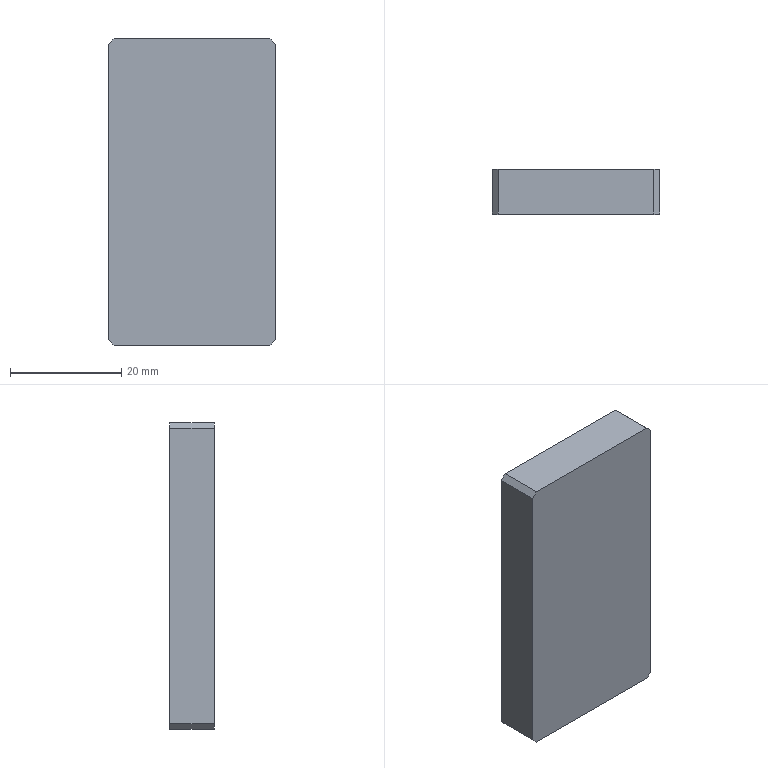Component | SolidWorks | GripperJaw1-1 | 1 solid | 16 faces | box 30 x 8 x 55 mm | volume 12147 mm3 | plane 14 | cylinder 2 | commonest cylinder face diameters 4 x2 | material 1060 Alloy
build123d program:
from build123d import *

# Parameters (mm, degrees)
SKETCH1_W           = 30
SKETCH1_H           = 55
BOSS_EXTRUDE1_DEPTH = 8
SKETCH2_W           = 20
SKETCH2_H           = 52
CUT_EXTRUDE1_DEPTH  = 2
FILLET1_R           = 2
CHAMFER1_SIZE       = 1


with BuildPart() as part:
    # Sketch1 → Boss-Extrude1 (new body)
    with BuildSketch(Plane.XY):
        Rectangle(SKETCH1_W, SKETCH1_H)
    extrude(amount=BOSS_EXTRUDE1_DEPTH)

    # Sketch2 → Cut-Extrude1 (cut)
    with BuildSketch(Plane.XY.offset(8)):
        with Locations((0, 27.5)):
            Rectangle(SKETCH2_W, SKETCH2_H)
    extrude(amount=-CUT_EXTRUDE1_DEPTH, mode=Mode.SUBTRACT)

    # Fillet1
    fillet1_edges = [part.edges().sort_by_distance(p)[0] for p in [
        (-10, 1.5, 7),
        (10, 1.5, 7),
    ]]
    fillet(fillet1_edges, radius=FILLET1_R)

    # Chamfer1
    chamfer1_edges = [part.edges().sort_by_distance(p)[0] for p in [
        (15, -27.5, 4),
        (-15, -27.5, 4),
        (-15, 27.5, 4),
        (15, 27.5, 4),
    ]]
    chamfer(chamfer1_edges, length=CHAMFER1_SIZE)


solid = part.part

# Placed as in the assembly
solid = solid.moved(Location((-45.188, -69.343, 163.22), (-90, 0, 0)))
STEP:
#1=COLOUR_RGB('',0.7922,0.8196,0.9333);
#2=FILL_AREA_STYLE_COLOUR('',#1);
#3=FILL_AREA_STYLE('',(#2));
#4=SURFACE_STYLE_FILL_AREA(#3);
#5=SURFACE_SIDE_STYLE('',(#4));
#6=SURFACE_STYLE_USAGE(.BOTH.,#5);
#7=PRESENTATION_STYLE_ASSIGNMENT((#6));
#8=CARTESIAN_POINT('',(-1.188,-2.415,7.469));
#9=VERTEX_POINT('',#8);
#10=CARTESIAN_POINT('',(-1.188,-2.415,5.383));
#11=VERTEX_POINT('',#10);
#12=CARTESIAN_POINT('',(-1.188,-2.415,5.343));
#13=DIRECTION('',(-0.,0.,-1.));
#14=VECTOR('',#13,39.37);
#15=LINE('',#12,#14);
#16=EDGE_CURVE('',#9,#11,#15,.T.);
#17=ORIENTED_EDGE('',*,*,#16,.F.);
#18=CARTESIAN_POINT('',(-1.188,-2.73,7.469));
#19=VERTEX_POINT('',#18);
#20=CARTESIAN_POINT('',(-1.188,-2.415,7.469));
#21=DIRECTION('',(0.,-1.,0.));
#22=VECTOR('',#21,39.37);
#23=LINE('',#20,#22);
#24=EDGE_CURVE('',#9,#19,#23,.T.);
#25=ORIENTED_EDGE('',*,*,#24,.T.);
#26=CARTESIAN_POINT('',(-1.188,-2.73,5.383));
#27=VERTEX_POINT('',#26);
#28=CARTESIAN_POINT('',(-1.188,-2.73,5.343));
#29=DIRECTION('',(-0.,0.,-1.));
#30=VECTOR('',#29,39.37);
#31=LINE('',#28,#30);
#32=EDGE_CURVE('',#19,#27,#31,.T.);
#33=ORIENTED_EDGE('',*,*,#32,.T.);
#34=CARTESIAN_POINT('',(-1.188,-2.415,5.383));
#35=DIRECTION('',(0.,1.,0.));
#36=VECTOR('',#35,39.37);
#37=LINE('',#34,#36);
#38=EDGE_CURVE('',#27,#11,#37,.T.);
#39=ORIENTED_EDGE('',*,*,#38,.T.);
#40=EDGE_LOOP('',(#17,#25,#33,#39));
#41=FACE_OUTER_BOUND('',#40,.T.);
#42=CARTESIAN_POINT('',(-1.188,-2.415,5.343));
#43=DIRECTION('',(-1.,0.,0.));
#44=DIRECTION('',(0.,0.,1.));
#45=AXIS2_PLACEMENT_3D('',#42,#43,#44);
#46=PLANE('',#45);
#47=ADVANCED_FACE('',(#41),#46,.F.);
#48=CARTESIAN_POINT('',(-1.228,-2.415,5.343));
#49=VERTEX_POINT('',#48);
#50=CARTESIAN_POINT('',(-1.385,-2.415,5.343));
#51=VERTEX_POINT('',#50);
#52=CARTESIAN_POINT('',(-2.37,-2.415,5.343));
#53=DIRECTION('',(-1.,0.,0.));
#54=VECTOR('',#53,39.37);
#55=LINE('',#52,#54);
#56=EDGE_CURVE('',#49,#51,#55,.T.);
#57=ORIENTED_EDGE('',*,*,#56,.F.);
#58=CARTESIAN_POINT('',(-1.228,-2.73,5.343));
#59=VERTEX_POINT('',#58);
#60=CARTESIAN_POINT('',(-1.228,-2.415,5.343));
#61=DIRECTION('',(0.,-1.,0.));
#62=VECTOR('',#61,39.37);
#63=LINE('',#60,#62);
#64=EDGE_CURVE('',#49,#59,#63,.T.);
#65=ORIENTED_EDGE('',*,*,#64,.T.);
#66=CARTESIAN_POINT('',(-2.33,-2.73,5.343));
#67=VERTEX_POINT('',#66);
#68=CARTESIAN_POINT('',(-2.37,-2.73,5.343));
#69=DIRECTION('',(-1.,0.,0.));
#70=VECTOR('',#69,39.37);
#71=LINE('',#68,#70);
#72=EDGE_CURVE('',#59,#67,#71,.T.);
#73=ORIENTED_EDGE('',*,*,#72,.T.);
#74=CARTESIAN_POINT('',(-2.33,-2.415,5.343));
#75=VERTEX_POINT('',#74);
#76=CARTESIAN_POINT('',(-2.33,-2.415,5.343));
#77=DIRECTION('',(0.,1.,0.));
#78=VECTOR('',#77,39.37);
#79=LINE('',#76,#78);
#80=EDGE_CURVE('',#67,#75,#79,.T.);
#81=ORIENTED_EDGE('',*,*,#80,.T.);
#82=CARTESIAN_POINT('',(-2.173,-2.415,5.343));
#83=VERTEX_POINT('',#82);
#84=CARTESIAN_POINT('',(-2.37,-2.415,5.343));
#85=DIRECTION('',(-1.,0.,0.));
#86=VECTOR('',#85,39.37);
#87=LINE('',#84,#86);
#88=EDGE_CURVE('',#83,#75,#87,.T.);
#89=ORIENTED_EDGE('',*,*,#88,.F.);
#90=CARTESIAN_POINT('',(-2.173,-2.494,5.343));
#91=VERTEX_POINT('',#90);
#92=CARTESIAN_POINT('',(-2.173,-2.415,5.343));
#93=DIRECTION('',(0.,-1.,0.));
#94=VECTOR('',#93,39.37);
#95=LINE('',#92,#94);
#96=EDGE_CURVE('',#83,#91,#95,.T.);
#97=ORIENTED_EDGE('',*,*,#96,.T.);
#98=CARTESIAN_POINT('',(-1.385,-2.494,5.343));
#99=VERTEX_POINT('',#98);
#100=CARTESIAN_POINT('',(-2.37,-2.494,5.343));
#101=DIRECTION('',(-1.,0.,0.));
#102=VECTOR('',#101,39.37);
#103=LINE('',#100,#102);
#104=EDGE_CURVE('',#99,#91,#103,.T.);
#105=ORIENTED_EDGE('',*,*,#104,.F.);
#106=CARTESIAN_POINT('',(-1.385,-2.415,5.343));
#107=DIRECTION('',(0.,1.,0.));
#108=VECTOR('',#107,39.37);
#109=LINE('',#106,#108);
#110=EDGE_CURVE('',#99,#51,#109,.T.);
#111=ORIENTED_EDGE('',*,*,#110,.T.);
#112=EDGE_LOOP('',(#57,#65,#73,#81,#89,#97,#105,#111));
#113=FACE_OUTER_BOUND('',#112,.T.);
#114=CARTESIAN_POINT('',(-2.37,-2.415,5.343));
#115=DIRECTION('',(0.,0.,1.));
#116=DIRECTION('',(0.,-1.,0.));
#117=AXIS2_PLACEMENT_3D('',#114,#115,#116);
#118=PLANE('',#117);
#119=ADVANCED_FACE('',(#113),#118,.F.);
#120=CARTESIAN_POINT('',(-2.37,-2.73,5.383));
#121=VERTEX_POINT('',#120);
#122=CARTESIAN_POINT('',(-2.37,-2.73,7.469));
#123=VERTEX_POINT('',#122);
#124=CARTESIAN_POINT('',(-2.37,-2.73,5.343));
#125=DIRECTION('',(0.,0.,1.));
#126=VECTOR('',#125,39.37);
#127=LINE('',#124,#126);
#128=EDGE_CURVE('',#121,#123,#127,.T.);
#129=ORIENTED_EDGE('',*,*,#128,.T.);
#130=CARTESIAN_POINT('',(-2.37,-2.415,7.469));
#131=VERTEX_POINT('',#130);
#132=CARTESIAN_POINT('',(-2.37,-2.415,7.469));
#133=DIRECTION('',(0.,1.,0.));
#134=VECTOR('',#133,39.37);
#135=LINE('',#132,#134);
#136=EDGE_CURVE('',#123,#131,#135,.T.);
#137=ORIENTED_EDGE('',*,*,#136,.T.);
#138=CARTESIAN_POINT('',(-2.37,-2.415,5.383));
#139=VERTEX_POINT('',#138);
#140=CARTESIAN_POINT('',(-2.37,-2.415,5.343));
#141=DIRECTION('',(0.,0.,1.));
#142=VECTOR('',#141,39.37);
#143=LINE('',#140,#142);
#144=EDGE_CURVE('',#139,#131,#143,.T.);
#145=ORIENTED_EDGE('',*,*,#144,.F.);
#146=CARTESIAN_POINT('',(-2.37,-2.415,5.383));
#147=DIRECTION('',(0.,-1.,0.));
#148=VECTOR('',#147,39.37);
#149=LINE('',#146,#148);
#150=EDGE_CURVE('',#139,#121,#149,.T.);
#151=ORIENTED_EDGE('',*,*,#150,.T.);
#152=EDGE_LOOP('',(#129,#137,#145,#151));
#153=FACE_OUTER_BOUND('',#152,.T.);
#154=CARTESIAN_POINT('',(-2.37,-2.415,5.343));
#155=DIRECTION('',(1.,0.,-0.));
#156=DIRECTION('',(-0.,0.,-1.));
#157=AXIS2_PLACEMENT_3D('',#154,#155,#156);
#158=PLANE('',#157);
#159=ADVANCED_FACE('',(#153),#158,.F.);
#160=CARTESIAN_POINT('',(-2.33,-2.73,7.509));
#161=VERTEX_POINT('',#160);
#162=CARTESIAN_POINT('',(-1.228,-2.73,7.509));
#163=VERTEX_POINT('',#162);
#164=CARTESIAN_POINT('',(-2.37,-2.73,7.509));
#165=DIRECTION('',(1.,0.,0.));
#166=VECTOR('',#165,39.37);
#167=LINE('',#164,#166);
#168=EDGE_CURVE('',#161,#163,#167,.T.);
#169=ORIENTED_EDGE('',*,*,#168,.T.);
#170=CARTESIAN_POINT('',(-1.228,-2.415,7.509));
#171=VERTEX_POINT('',#170);
#172=CARTESIAN_POINT('',(-1.228,-2.415,7.509));
#173=DIRECTION('',(0.,1.,0.));
#174=VECTOR('',#173,39.37);
#175=LINE('',#172,#174);
#176=EDGE_CURVE('',#163,#171,#175,.T.);
#177=ORIENTED_EDGE('',*,*,#176,.T.);
#178=CARTESIAN_POINT('',(-2.33,-2.415,7.509));
#179=VERTEX_POINT('',#178);
#180=CARTESIAN_POINT('',(-2.37,-2.415,7.509));
#181=DIRECTION('',(1.,0.,0.));
#182=VECTOR('',#181,39.37);
#183=LINE('',#180,#182);
#184=EDGE_CURVE('',#179,#171,#183,.T.);
#185=ORIENTED_EDGE('',*,*,#184,.F.);
#186=CARTESIAN_POINT('',(-2.33,-2.415,7.509));
#187=DIRECTION('',(0.,-1.,0.));
#188=VECTOR('',#187,39.37);
#189=LINE('',#186,#188);
#190=EDGE_CURVE('',#179,#161,#189,.T.);
#191=ORIENTED_EDGE('',*,*,#190,.T.);
#192=EDGE_LOOP('',(#169,#177,#185,#191));
#193=FACE_OUTER_BOUND('',#192,.T.);
#194=CARTESIAN_POINT('',(-2.37,-2.415,7.509));
#195=DIRECTION('',(0.,0.,-1.));
#196=DIRECTION('',(0.,1.,0.));
#197=AXIS2_PLACEMENT_3D('',#194,#195,#196);
#198=PLANE('',#197);
#199=ADVANCED_FACE('',(#193),#198,.F.);
#200=ORIENTED_EDGE('',*,*,#184,.T.);
#201=CARTESIAN_POINT('',(-0.9621,-2.415,7.243));
#202=DIRECTION('',(0.7071,0.,-0.7071));
#203=VECTOR('',#202,39.37);
#204=LINE('',#201,#203);
#205=EDGE_CURVE('',#171,#9,#204,.T.);
#206=ORIENTED_EDGE('',*,*,#205,.T.);
#207=ORIENTED_EDGE('',*,*,#16,.T.);
#208=CARTESIAN_POINT('',(-0.9621,-2.415,5.609));
#209=DIRECTION('',(-0.7071,0.,-0.7071));
#210=VECTOR('',#209,39.37);
#211=LINE('',#208,#210);
#212=EDGE_CURVE('',#11,#49,#211,.T.);
#213=ORIENTED_EDGE('',*,*,#212,.T.);
#214=ORIENTED_EDGE('',*,*,#56,.T.);
#215=CARTESIAN_POINT('',(-1.385,-2.415,6.288));
#216=VERTEX_POINT('',#215);
#217=CARTESIAN_POINT('',(-1.385,-2.415,4.32));
#218=DIRECTION('',(-0.,0.,-1.));
#219=VECTOR('',#218,39.37);
#220=LINE('',#217,#219);
#221=EDGE_CURVE('',#216,#51,#220,.T.);
#222=ORIENTED_EDGE('',*,*,#221,.F.);
#223=CARTESIAN_POINT('',(-1.464,-2.415,6.367));
#224=VERTEX_POINT('',#223);
#225=CARTESIAN_POINT('',(-1.464,-2.415,6.288));
#226=DIRECTION('',(0.,-1.,0.));
#227=DIRECTION('',(1.,0.,0.));
#228=AXIS2_PLACEMENT_3D('',#225,#226,#227);
#229=CIRCLE('',#228,0.07874);
#230=EDGE_CURVE('',#216,#224,#229,.T.);
#231=ORIENTED_EDGE('',*,*,#230,.T.);
#232=CARTESIAN_POINT('',(-2.094,-2.415,6.367));
#233=VERTEX_POINT('',#232);
#234=CARTESIAN_POINT('',(-2.173,-2.415,6.367));
#235=DIRECTION('',(1.,0.,-0.));
#236=VECTOR('',#235,39.37);
#237=LINE('',#234,#236);
#238=EDGE_CURVE('',#233,#224,#237,.T.);
#239=ORIENTED_EDGE('',*,*,#238,.F.);
#240=CARTESIAN_POINT('',(-2.173,-2.415,6.288));
#241=VERTEX_POINT('',#240);
#242=CARTESIAN_POINT('',(-2.094,-2.415,6.288));
#243=DIRECTION('',(0.,-1.,0.));
#244=DIRECTION('',(1.,0.,0.));
#245=AXIS2_PLACEMENT_3D('',#242,#243,#244);
#246=CIRCLE('',#245,0.07874);
#247=EDGE_CURVE('',#233,#241,#246,.T.);
#248=ORIENTED_EDGE('',*,*,#247,.T.);
#249=CARTESIAN_POINT('',(-2.173,-2.415,6.426));
#250=DIRECTION('',(0.,0.,1.));
#251=VECTOR('',#250,39.37);
#252=LINE('',#249,#251);
#253=EDGE_CURVE('',#83,#241,#252,.T.);
#254=ORIENTED_EDGE('',*,*,#253,.F.);
#255=ORIENTED_EDGE('',*,*,#88,.T.);
#256=CARTESIAN_POINT('',(-2.596,-2.415,5.609));
#257=DIRECTION('',(-0.7071,0.,0.7071));
#258=VECTOR('',#257,39.37);
#259=LINE('',#256,#258);
#260=EDGE_CURVE('',#75,#139,#259,.T.);
#261=ORIENTED_EDGE('',*,*,#260,.T.);
#262=ORIENTED_EDGE('',*,*,#144,.T.);
#263=CARTESIAN_POINT('',(-2.596,-2.415,7.243));
#264=DIRECTION('',(0.7071,0.,0.7071));
#265=VECTOR('',#264,39.37);
#266=LINE('',#263,#265);
#267=EDGE_CURVE('',#131,#179,#266,.T.);
#268=ORIENTED_EDGE('',*,*,#267,.T.);
#269=EDGE_LOOP('',(#200,#206,#207,#213,#214,#222,#231,#239,#248,#254,#255,#261,#262,#268));
#270=FACE_OUTER_BOUND('',#269,.T.);
#271=CARTESIAN_POINT('',(-1.779,-2.415,6.426));
#272=DIRECTION('',(0.,1.,0.));
#273=DIRECTION('',(1.,0.,0.));
#274=AXIS2_PLACEMENT_3D('',#271,#272,#273);
#275=PLANE('',#274);
#276=ADVANCED_FACE('',(#270),#275,.T.);
#277=ORIENTED_EDGE('',*,*,#32,.F.);
#278=CARTESIAN_POINT('',(-1.188,-2.73,7.469));
#279=DIRECTION('',(-0.7071,0.,0.7071));
#280=VECTOR('',#279,39.37);
#281=LINE('',#278,#280);
#282=EDGE_CURVE('',#19,#163,#281,.T.);
#283=ORIENTED_EDGE('',*,*,#282,.T.);
#284=ORIENTED_EDGE('',*,*,#168,.F.);
#285=CARTESIAN_POINT('',(-2.33,-2.73,7.509));
#286=DIRECTION('',(-0.7071,0.,-0.7071));
#287=VECTOR('',#286,39.37);
#288=LINE('',#285,#287);
#289=EDGE_CURVE('',#161,#123,#288,.T.);
#290=ORIENTED_EDGE('',*,*,#289,.T.);
#291=ORIENTED_EDGE('',*,*,#128,.F.);
#292=CARTESIAN_POINT('',(-2.37,-2.73,5.383));
#293=DIRECTION('',(0.7071,0.,-0.7071));
#294=VECTOR('',#293,39.37);
#295=LINE('',#292,#294);
#296=EDGE_CURVE('',#121,#67,#295,.T.);
#297=ORIENTED_EDGE('',*,*,#296,.T.);
#298=ORIENTED_EDGE('',*,*,#72,.F.);
#299=CARTESIAN_POINT('',(-1.228,-2.73,5.343));
#300=DIRECTION('',(0.7071,0.,0.7071));
#301=VECTOR('',#300,39.37);
#302=LINE('',#299,#301);
#303=EDGE_CURVE('',#59,#27,#302,.T.);
#304=ORIENTED_EDGE('',*,*,#303,.T.);
#305=EDGE_LOOP('',(#277,#283,#284,#290,#291,#297,#298,#304));
#306=FACE_OUTER_BOUND('',#305,.T.);
#307=CARTESIAN_POINT('',(-1.779,-2.73,6.426));
#308=DIRECTION('',(0.,1.,0.));
#309=DIRECTION('',(1.,0.,0.));
#310=AXIS2_PLACEMENT_3D('',#307,#308,#309);
#311=PLANE('',#310);
#312=ADVANCED_FACE('',(#306),#311,.F.);
#313=CARTESIAN_POINT('',(-2.094,-2.494,6.367));
#314=VERTEX_POINT('',#313);
#315=CARTESIAN_POINT('',(-1.464,-2.494,6.367));
#316=VERTEX_POINT('',#315);
#317=CARTESIAN_POINT('',(-2.173,-2.494,6.367));
#318=DIRECTION('',(1.,0.,-0.));
#319=VECTOR('',#318,39.37);
#320=LINE('',#317,#319);
#321=EDGE_CURVE('',#314,#316,#320,.T.);
#322=ORIENTED_EDGE('',*,*,#321,.T.);
#323=CARTESIAN_POINT('',(-1.385,-2.494,6.288));
#324=VERTEX_POINT('',#323);
#325=CARTESIAN_POINT('',(-1.464,-2.494,6.288));
#326=DIRECTION('',(0.,1.,0.));
#327=DIRECTION('',(1.,0.,0.));
#328=AXIS2_PLACEMENT_3D('',#325,#326,#327);
#329=CIRCLE('',#328,0.07874);
#330=EDGE_CURVE('',#316,#324,#329,.T.);
#331=ORIENTED_EDGE('',*,*,#330,.T.);
#332=CARTESIAN_POINT('',(-1.385,-2.494,4.32));
#333=DIRECTION('',(-0.,0.,-1.));
#334=VECTOR('',#333,39.37);
#335=LINE('',#332,#334);
#336=EDGE_CURVE('',#324,#99,#335,.T.);
#337=ORIENTED_EDGE('',*,*,#336,.T.);
#338=ORIENTED_EDGE('',*,*,#104,.T.);
#339=CARTESIAN_POINT('',(-2.173,-2.494,6.288));
#340=VERTEX_POINT('',#339);
#341=CARTESIAN_POINT('',(-2.173,-2.494,4.32));
#342=DIRECTION('',(0.,0.,1.));
#343=VECTOR('',#342,39.37);
#344=LINE('',#341,#343);
#345=EDGE_CURVE('',#91,#340,#344,.T.);
#346=ORIENTED_EDGE('',*,*,#345,.T.);
#347=CARTESIAN_POINT('',(-2.094,-2.494,6.288));
#348=DIRECTION('',(0.,1.,0.));
#349=DIRECTION('',(1.,0.,0.));
#350=AXIS2_PLACEMENT_3D('',#347,#348,#349);
#351=CIRCLE('',#350,0.07874);
#352=EDGE_CURVE('',#340,#314,#351,.T.);
#353=ORIENTED_EDGE('',*,*,#352,.T.);
#354=EDGE_LOOP('',(#322,#331,#337,#338,#346,#353));
#355=FACE_OUTER_BOUND('',#354,.T.);
#356=CARTESIAN_POINT('',(-1.779,-2.494,6.426));
#357=DIRECTION('',(0.,1.,0.));
#358=DIRECTION('',(1.,0.,0.));
#359=AXIS2_PLACEMENT_3D('',#356,#357,#358);
#360=PLANE('',#359);
#361=ADVANCED_FACE('',(#355),#360,.T.);
#362=ORIENTED_EDGE('',*,*,#336,.F.);
#363=CARTESIAN_POINT('',(-1.385,-2.415,6.288));
#364=DIRECTION('',(0.,1.,0.));
#365=VECTOR('',#364,39.37);
#366=LINE('',#363,#365);
#367=EDGE_CURVE('',#324,#216,#366,.T.);
#368=ORIENTED_EDGE('',*,*,#367,.T.);
#369=ORIENTED_EDGE('',*,*,#221,.T.);
#370=ORIENTED_EDGE('',*,*,#110,.F.);
#371=EDGE_LOOP('',(#362,#368,#369,#370));
#372=FACE_OUTER_BOUND('',#371,.T.);
#373=CARTESIAN_POINT('',(-1.385,-2.494,4.32));
#374=DIRECTION('',(1.,0.,-0.));
#375=DIRECTION('',(-0.,0.,-1.));
#376=AXIS2_PLACEMENT_3D('',#373,#374,#375);
#377=PLANE('',#376);
#378=ADVANCED_FACE('',(#372),#377,.F.);
#379=ORIENTED_EDGE('',*,*,#253,.T.);
#380=CARTESIAN_POINT('',(-2.173,-2.494,6.288));
#381=DIRECTION('',(0.,-1.,0.));
#382=VECTOR('',#381,39.37);
#383=LINE('',#380,#382);
#384=EDGE_CURVE('',#241,#340,#383,.T.);
#385=ORIENTED_EDGE('',*,*,#384,.T.);
#386=ORIENTED_EDGE('',*,*,#345,.F.);
#387=ORIENTED_EDGE('',*,*,#96,.F.);
#388=EDGE_LOOP('',(#379,#385,#386,#387));
#389=FACE_OUTER_BOUND('',#388,.T.);
#390=CARTESIAN_POINT('',(-2.173,-2.494,4.32));
#391=DIRECTION('',(-1.,0.,0.));
#392=DIRECTION('',(0.,1.,0.));
#393=AXIS2_PLACEMENT_3D('',#390,#391,#392);
#394=PLANE('',#393);
#395=ADVANCED_FACE('',(#389),#394,.F.);
#396=ORIENTED_EDGE('',*,*,#238,.T.);
#397=CARTESIAN_POINT('',(-1.464,-2.494,6.367));
#398=DIRECTION('',(0.,-1.,0.));
#399=VECTOR('',#398,39.37);
#400=LINE('',#397,#399);
#401=EDGE_CURVE('',#224,#316,#400,.T.);
#402=ORIENTED_EDGE('',*,*,#401,.T.);
#403=ORIENTED_EDGE('',*,*,#321,.F.);
#404=CARTESIAN_POINT('',(-2.094,-2.415,6.367));
#405=DIRECTION('',(0.,1.,0.));
#406=VECTOR('',#405,39.37);
#407=LINE('',#404,#406);
#408=EDGE_CURVE('',#314,#233,#407,.T.);
#409=ORIENTED_EDGE('',*,*,#408,.T.);
#410=EDGE_LOOP('',(#396,#402,#403,#409));
#411=FACE_OUTER_BOUND('',#410,.T.);
#412=CARTESIAN_POINT('',(-2.173,-2.494,6.367));
#413=DIRECTION('',(0.,0.,1.));
#414=DIRECTION('',(1.,0.,-0.));
#415=AXIS2_PLACEMENT_3D('',#412,#413,#414);
#416=PLANE('',#415);
#417=ADVANCED_FACE('',(#411),#416,.F.);
#418=ORIENTED_EDGE('',*,*,#330,.F.);
#419=ORIENTED_EDGE('',*,*,#401,.F.);
#420=ORIENTED_EDGE('',*,*,#230,.F.);
#421=ORIENTED_EDGE('',*,*,#367,.F.);
#422=EDGE_LOOP('',(#418,#419,#420,#421));
#423=FACE_OUTER_BOUND('',#422,.T.);
#424=CARTESIAN_POINT('',(-1.464,-2.494,6.288));
#425=DIRECTION('',(0.,-1.,0.));
#426=DIRECTION('',(-1.,0.,0.));
#427=AXIS2_PLACEMENT_3D('',#424,#425,#426);
#428=CYLINDRICAL_SURFACE('',#427,0.07874);
#429=ADVANCED_FACE('',(#423),#428,.F.);
#430=ORIENTED_EDGE('',*,*,#352,.F.);
#431=ORIENTED_EDGE('',*,*,#384,.F.);
#432=ORIENTED_EDGE('',*,*,#247,.F.);
#433=ORIENTED_EDGE('',*,*,#408,.F.);
#434=EDGE_LOOP('',(#430,#431,#432,#433));
#435=FACE_OUTER_BOUND('',#434,.T.);
#436=CARTESIAN_POINT('',(-2.094,-2.494,6.288));
#437=DIRECTION('',(0.,-1.,0.));
#438=DIRECTION('',(-1.,0.,0.));
#439=AXIS2_PLACEMENT_3D('',#436,#437,#438);
#440=CYLINDRICAL_SURFACE('',#439,0.07874);
#441=ADVANCED_FACE('',(#435),#440,.F.);
#442=ORIENTED_EDGE('',*,*,#205,.F.);
#443=ORIENTED_EDGE('',*,*,#176,.F.);
#444=ORIENTED_EDGE('',*,*,#282,.F.);
#445=ORIENTED_EDGE('',*,*,#24,.F.);
#446=EDGE_LOOP('',(#442,#443,#444,#445));
#447=FACE_OUTER_BOUND('',#446,.T.);
#448=CARTESIAN_POINT('',(-1.188,-2.415,7.469));
#449=DIRECTION('',(-0.7071,0.,-0.7071));
#450=DIRECTION('',(0.,-1.,0.));
#451=AXIS2_PLACEMENT_3D('',#448,#449,#450);
#452=PLANE('',#451);
#453=ADVANCED_FACE('',(#447),#452,.F.);
#454=ORIENTED_EDGE('',*,*,#267,.F.);
#455=ORIENTED_EDGE('',*,*,#136,.F.);
#456=ORIENTED_EDGE('',*,*,#289,.F.);
#457=ORIENTED_EDGE('',*,*,#190,.F.);
#458=EDGE_LOOP('',(#454,#455,#456,#457));
#459=FACE_OUTER_BOUND('',#458,.T.);
#460=CARTESIAN_POINT('',(-2.33,-2.415,7.509));
#461=DIRECTION('',(0.7071,0.,-0.7071));
#462=DIRECTION('',(0.,-1.,0.));
#463=AXIS2_PLACEMENT_3D('',#460,#461,#462);
#464=PLANE('',#463);
#465=ADVANCED_FACE('',(#459),#464,.F.);
#466=ORIENTED_EDGE('',*,*,#212,.F.);
#467=ORIENTED_EDGE('',*,*,#38,.F.);
#468=ORIENTED_EDGE('',*,*,#303,.F.);
#469=ORIENTED_EDGE('',*,*,#64,.F.);
#470=EDGE_LOOP('',(#466,#467,#468,#469));
#471=FACE_OUTER_BOUND('',#470,.T.);
#472=CARTESIAN_POINT('',(-1.228,-2.415,5.343));
#473=DIRECTION('',(-0.7071,0.,0.7071));
#474=DIRECTION('',(0.,-1.,0.));
#475=AXIS2_PLACEMENT_3D('',#472,#473,#474);
#476=PLANE('',#475);
#477=ADVANCED_FACE('',(#471),#476,.F.);
#478=ORIENTED_EDGE('',*,*,#260,.F.);
#479=ORIENTED_EDGE('',*,*,#80,.F.);
#480=ORIENTED_EDGE('',*,*,#296,.F.);
#481=ORIENTED_EDGE('',*,*,#150,.F.);
#482=EDGE_LOOP('',(#478,#479,#480,#481));
#483=FACE_OUTER_BOUND('',#482,.T.);
#484=CARTESIAN_POINT('',(-2.37,-2.415,5.383));
#485=DIRECTION('',(0.7071,0.,0.7071));
#486=DIRECTION('',(0.,-1.,0.));
#487=AXIS2_PLACEMENT_3D('',#484,#485,#486);
#488=PLANE('',#487);
#489=ADVANCED_FACE('',(#483),#488,.F.);
#490=CLOSED_SHELL('',(#47,#119,#159,#199,#276,#312,#361,#378,#395,#417,#429,#441,#453,#465,#477,#489));
#491=MANIFOLD_SOLID_BREP('',#490);
#492=STYLED_ITEM('',(#7),#491);
#493=(LENGTH_UNIT()NAMED_UNIT(*)SI_UNIT($,.METRE.));
#494=LENGTH_MEASURE_WITH_UNIT(LENGTH_MEASURE(0.0254),#493);
#495=DIMENSIONAL_EXPONENTS(1.,0.,0.,0.,0.,0.,0.);
#496=(CONVERSION_BASED_UNIT('',#494)LENGTH_UNIT()NAMED_UNIT(#495));
#497=UNCERTAINTY_MEASURE_WITH_UNIT(LENGTH_MEASURE(0.00001),#496,'','');
#498=(NAMED_UNIT(*)PLANE_ANGLE_UNIT()SI_UNIT($,.RADIAN.));
#499=(NAMED_UNIT(*)SI_UNIT($,.STERADIAN.)SOLID_ANGLE_UNIT());
#500=(GEOMETRIC_REPRESENTATION_CONTEXT(3)GLOBAL_UNCERTAINTY_ASSIGNED_CONTEXT((#497))GLOBAL_UNIT_ASSIGNED_CONTEXT((#496,#498,#499))REPRESENTATION_CONTEXT('',''));
#501=MECHANICAL_DESIGN_GEOMETRIC_PRESENTATION_REPRESENTATION('',(#492),#500);
#502=PRESENTATION_LAYER_ASSIGNMENT('','',(#492));
#503=CARTESIAN_POINT('',(0.,0.,0.));
#504=DIRECTION('',(0.,0.,1.));
#505=DIRECTION('',(1.,0.,0.));
#506=AXIS2_PLACEMENT_3D('',#503,#504,#505);
#507=(LENGTH_UNIT()NAMED_UNIT(*)SI_UNIT($,.METRE.));
#508=LENGTH_MEASURE_WITH_UNIT(LENGTH_MEASURE(0.0254),#507);
#509=DIMENSIONAL_EXPONENTS(1.,0.,0.,0.,0.,0.,0.);
#510=(CONVERSION_BASED_UNIT('',#508)LENGTH_UNIT()NAMED_UNIT(#509));
#511=UNCERTAINTY_MEASURE_WITH_UNIT(LENGTH_MEASURE(0.00001),#510,'','');
#512=(NAMED_UNIT(*)PLANE_ANGLE_UNIT()SI_UNIT($,.RADIAN.));
#513=(NAMED_UNIT(*)SI_UNIT($,.STERADIAN.)SOLID_ANGLE_UNIT());
#514=(GEOMETRIC_REPRESENTATION_CONTEXT(3)GLOBAL_UNCERTAINTY_ASSIGNED_CONTEXT((#511))GLOBAL_UNIT_ASSIGNED_CONTEXT((#510,#512,#513))REPRESENTATION_CONTEXT('',''));
#515=ADVANCED_BREP_SHAPE_REPRESENTATION('',(#491,#506),#514);